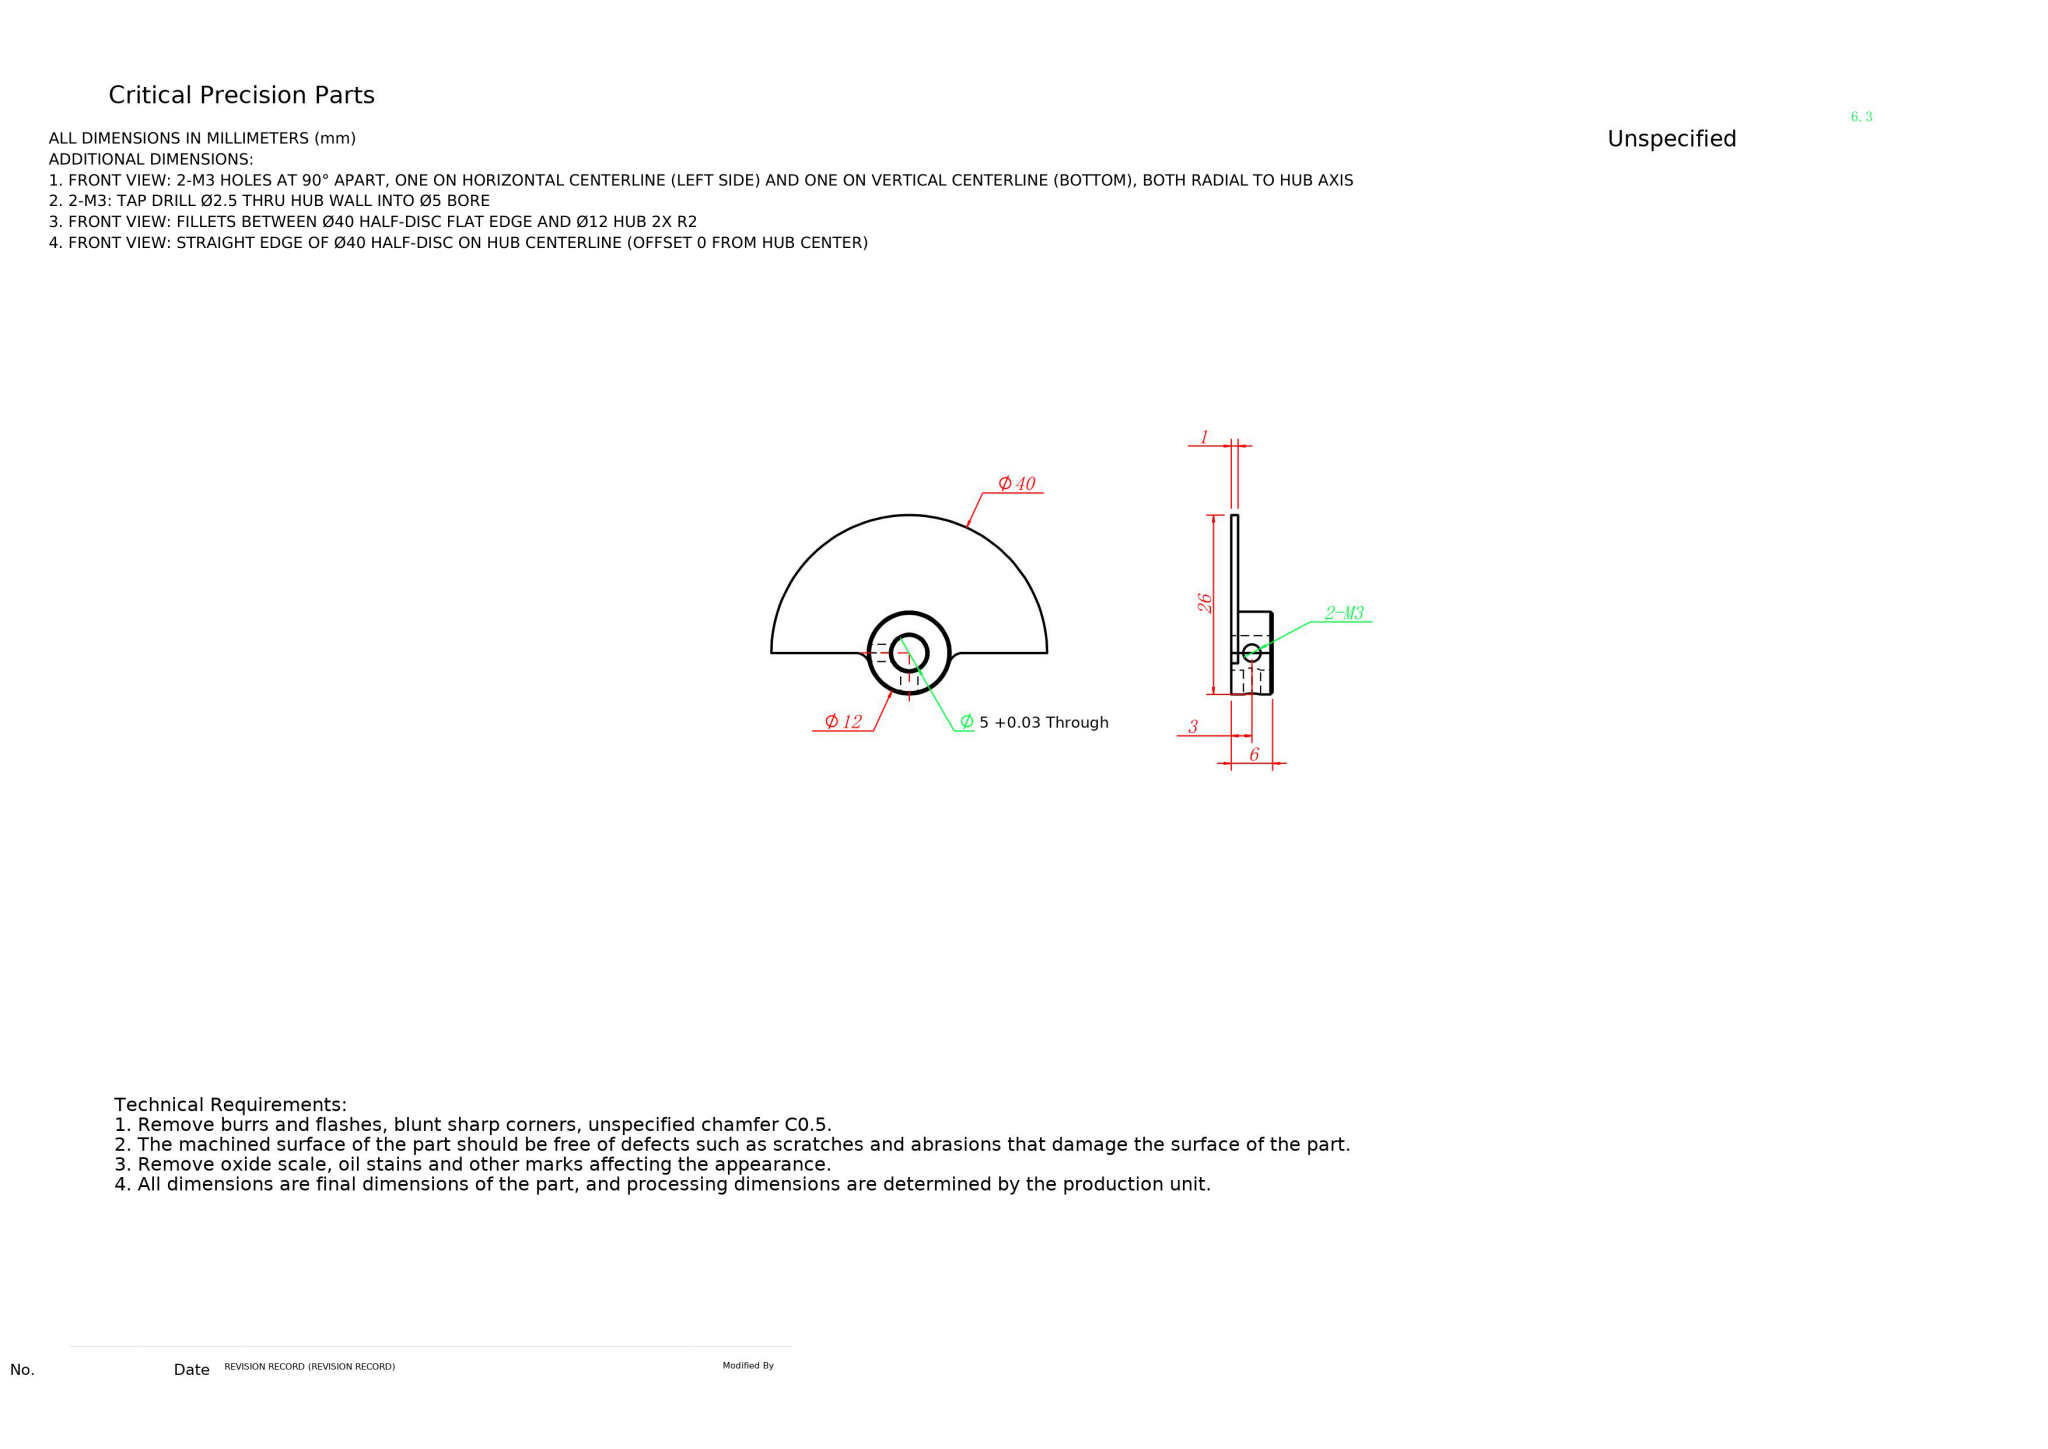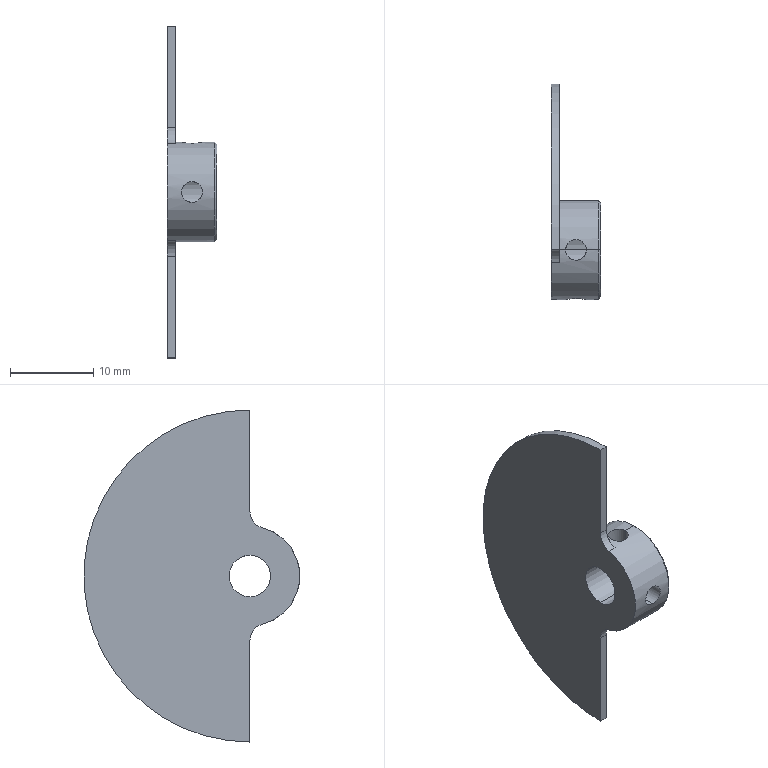Part | NX | mm | 1 solid | 22 faces | box 6 x 26 x 40 mm | volume 1096 mm3 | cylinder 13 | plane 5 | cone 4 | commonest cylinder face diameters 2.5 x4 1 x2 5 x2 12 x2 4 x2 40 x1
STEP:
#1=COLOUR_RGB('',0.7922,0.8196,0.9333);
#2=FILL_AREA_STYLE_COLOUR('',#1);
#3=FILL_AREA_STYLE('',(#2));
#4=SURFACE_STYLE_FILL_AREA(#3);
#5=SURFACE_SIDE_STYLE('',(#4));
#6=SURFACE_STYLE_USAGE(.BOTH.,#5);
#7=PRESENTATION_STYLE_ASSIGNMENT((#6));
#8=CARTESIAN_POINT('',(0.5,0.00003908,20.));
#9=VERTEX_POINT('',#8);
#10=CARTESIAN_POINT('',(0.5,-0.,19.994));
#11=VERTEX_POINT('',#10);
#12=CARTESIAN_POINT('',(0.5,0.5,19.994));
#13=DIRECTION('',(1.,0.,0.));
#14=DIRECTION('',(0.,0.,-1.));
#15=AXIS2_PLACEMENT_3D('',#12,#13,#14);
#16=CIRCLE('',#15,0.5);
#17=EDGE_CURVE('',#9,#11,#16,.T.);
#18=ORIENTED_EDGE('',*,*,#17,.F.);
#19=CARTESIAN_POINT('',(-0.5,0.00003908,20.));
#20=VERTEX_POINT('',#19);
#21=CARTESIAN_POINT('',(-0.0000125,0.00003908,20.));
#22=DIRECTION('',(-1.,0.,0.));
#23=VECTOR('',#22,1000.);
#24=LINE('',#21,#23);
#25=EDGE_CURVE('',#9,#20,#24,.T.);
#26=ORIENTED_EDGE('',*,*,#25,.T.);
#27=CARTESIAN_POINT('',(-0.5,-0.,19.994));
#28=VERTEX_POINT('',#27);
#29=CARTESIAN_POINT('',(-0.5,0.5,19.994));
#30=DIRECTION('',(-1.,0.,0.));
#31=DIRECTION('',(0.,0.,-1.));
#32=AXIS2_PLACEMENT_3D('',#29,#30,#31);
#33=CIRCLE('',#32,0.5);
#34=EDGE_CURVE('',#28,#20,#33,.T.);
#35=ORIENTED_EDGE('',*,*,#34,.F.);
#36=CARTESIAN_POINT('',(-0.5,-0.,19.994));
#37=DIRECTION('',(-1.,0.,0.));
#38=VECTOR('',#37,1000.);
#39=LINE('',#36,#38);
#40=EDGE_CURVE('',#11,#28,#39,.T.);
#41=ORIENTED_EDGE('',*,*,#40,.F.);
#42=EDGE_LOOP('',(#18,#26,#35,#41));
#43=FACE_OUTER_BOUND('',#42,.T.);
#44=CARTESIAN_POINT('',(0.5,0.5,19.994));
#45=DIRECTION('',(-1.,0.,0.));
#46=DIRECTION('',(0.,0.,1.));
#47=AXIS2_PLACEMENT_3D('',#44,#45,#46);
#48=CYLINDRICAL_SURFACE('',#47,0.5);
#49=ADVANCED_FACE('',(#43),#48,.T.);
#50=CARTESIAN_POINT('',(0.5,-0.,-19.994));
#51=VERTEX_POINT('',#50);
#52=CARTESIAN_POINT('',(0.5,0.00003908,-20.));
#53=VERTEX_POINT('',#52);
#54=CARTESIAN_POINT('',(0.5,0.5,-19.994));
#55=DIRECTION('',(1.,0.,0.));
#56=DIRECTION('',(0.,0.,-1.));
#57=AXIS2_PLACEMENT_3D('',#54,#55,#56);
#58=CIRCLE('',#57,0.5);
#59=EDGE_CURVE('',#51,#53,#58,.T.);
#60=ORIENTED_EDGE('',*,*,#59,.T.);
#61=CARTESIAN_POINT('',(0.5,0.,0.));
#62=DIRECTION('',(1.,0.,0.));
#63=DIRECTION('',(0.,0.,-1.));
#64=AXIS2_PLACEMENT_3D('',#61,#62,#63);
#65=CIRCLE('',#64,20.);
#66=EDGE_CURVE('',#53,#9,#65,.T.);
#67=ORIENTED_EDGE('',*,*,#66,.T.);
#68=ORIENTED_EDGE('',*,*,#17,.T.);
#69=CARTESIAN_POINT('',(0.5,-0.,7.746));
#70=VERTEX_POINT('',#69);
#71=CARTESIAN_POINT('',(0.5,0.,6.));
#72=DIRECTION('',(0.,-0.,1.));
#73=VECTOR('',#72,1000.);
#74=LINE('',#71,#73);
#75=EDGE_CURVE('',#70,#11,#74,.T.);
#76=ORIENTED_EDGE('',*,*,#75,.F.);
#77=CARTESIAN_POINT('',(0.5,-1.5,5.809));
#78=VERTEX_POINT('',#77);
#79=CARTESIAN_POINT('',(0.5,-2.,7.746));
#80=DIRECTION('',(-1.,0.,0.));
#81=DIRECTION('',(0.,0.,-1.));
#82=AXIS2_PLACEMENT_3D('',#79,#80,#81);
#83=CIRCLE('',#82,2.);
#84=EDGE_CURVE('',#70,#78,#83,.T.);
#85=ORIENTED_EDGE('',*,*,#84,.T.);
#86=CARTESIAN_POINT('',(0.5,0.,6.));
#87=VERTEX_POINT('',#86);
#88=CARTESIAN_POINT('',(0.5,0.,0.));
#89=DIRECTION('',(1.,0.,0.));
#90=DIRECTION('',(0.,0.,-1.));
#91=AXIS2_PLACEMENT_3D('',#88,#89,#90);
#92=CIRCLE('',#91,6.);
#93=EDGE_CURVE('',#87,#78,#92,.T.);
#94=ORIENTED_EDGE('',*,*,#93,.F.);
#95=CARTESIAN_POINT('',(0.5,0.,-6.));
#96=VERTEX_POINT('',#95);
#97=CARTESIAN_POINT('',(0.5,0.,0.));
#98=DIRECTION('',(1.,0.,0.));
#99=DIRECTION('',(0.,0.,-1.));
#100=AXIS2_PLACEMENT_3D('',#97,#98,#99);
#101=CIRCLE('',#100,6.);
#102=EDGE_CURVE('',#96,#87,#101,.T.);
#103=ORIENTED_EDGE('',*,*,#102,.F.);
#104=CARTESIAN_POINT('',(0.5,-1.5,-5.809));
#105=VERTEX_POINT('',#104);
#106=CARTESIAN_POINT('',(0.5,0.,0.));
#107=DIRECTION('',(1.,0.,0.));
#108=DIRECTION('',(0.,0.,-1.));
#109=AXIS2_PLACEMENT_3D('',#106,#107,#108);
#110=CIRCLE('',#109,6.);
#111=EDGE_CURVE('',#105,#96,#110,.T.);
#112=ORIENTED_EDGE('',*,*,#111,.F.);
#113=CARTESIAN_POINT('',(0.5,-0.,-7.746));
#114=VERTEX_POINT('',#113);
#115=CARTESIAN_POINT('',(0.5,-2.,-7.746));
#116=DIRECTION('',(-1.,0.,0.));
#117=DIRECTION('',(0.,0.,-1.));
#118=AXIS2_PLACEMENT_3D('',#115,#116,#117);
#119=CIRCLE('',#118,2.);
#120=EDGE_CURVE('',#105,#114,#119,.T.);
#121=ORIENTED_EDGE('',*,*,#120,.T.);
#122=CARTESIAN_POINT('',(0.5,-0.,-20.5));
#123=DIRECTION('',(0.,0.,1.));
#124=VECTOR('',#123,1000.);
#125=LINE('',#122,#124);
#126=EDGE_CURVE('',#51,#114,#125,.T.);
#127=ORIENTED_EDGE('',*,*,#126,.F.);
#128=EDGE_LOOP('',(#60,#67,#68,#76,#85,#94,#103,#112,#121,#127));
#129=FACE_OUTER_BOUND('',#128,.T.);
#130=CARTESIAN_POINT('',(0.5,0.,0.));
#131=DIRECTION('',(1.,0.,0.));
#132=DIRECTION('',(0.,1.,0.));
#133=AXIS2_PLACEMENT_3D('',#130,#131,#132);
#134=PLANE('',#133);
#135=ADVANCED_FACE('',(#129),#134,.T.);
#136=CARTESIAN_POINT('',(-0.5,0.,-2.5));
#137=VERTEX_POINT('',#136);
#138=CARTESIAN_POINT('',(-0.5,0.,2.5));
#139=VERTEX_POINT('',#138);
#140=CARTESIAN_POINT('',(-0.5,0.,0.));
#141=DIRECTION('',(1.,0.,0.));
#142=DIRECTION('',(0.,0.,-1.));
#143=AXIS2_PLACEMENT_3D('',#140,#141,#142);
#144=CIRCLE('',#143,2.5);
#145=EDGE_CURVE('',#137,#139,#144,.T.);
#146=ORIENTED_EDGE('',*,*,#145,.T.);
#147=CARTESIAN_POINT('',(-0.5,0.,0.));
#148=DIRECTION('',(1.,0.,0.));
#149=DIRECTION('',(0.,0.,-1.));
#150=AXIS2_PLACEMENT_3D('',#147,#148,#149);
#151=CIRCLE('',#150,2.5);
#152=EDGE_CURVE('',#139,#137,#151,.T.);
#153=ORIENTED_EDGE('',*,*,#152,.T.);
#154=EDGE_LOOP('',(#146,#153));
#155=FACE_BOUND('',#154,.T.);
#156=CARTESIAN_POINT('',(-0.5,0.00003908,-20.));
#157=VERTEX_POINT('',#156);
#158=CARTESIAN_POINT('',(-0.5,0.,0.));
#159=DIRECTION('',(1.,0.,0.));
#160=DIRECTION('',(0.,0.,-1.));
#161=AXIS2_PLACEMENT_3D('',#158,#159,#160);
#162=CIRCLE('',#161,20.);
#163=EDGE_CURVE('',#157,#20,#162,.T.);
#164=ORIENTED_EDGE('',*,*,#163,.F.);
#165=CARTESIAN_POINT('',(-0.5,-0.,-19.994));
#166=VERTEX_POINT('',#165);
#167=CARTESIAN_POINT('',(-0.5,0.5,-19.994));
#168=DIRECTION('',(-1.,0.,0.));
#169=DIRECTION('',(0.,0.,-1.));
#170=AXIS2_PLACEMENT_3D('',#167,#168,#169);
#171=CIRCLE('',#170,0.5);
#172=EDGE_CURVE('',#157,#166,#171,.T.);
#173=ORIENTED_EDGE('',*,*,#172,.T.);
#174=CARTESIAN_POINT('',(-0.5,-0.,-7.746));
#175=VERTEX_POINT('',#174);
#176=CARTESIAN_POINT('',(-0.5,-0.,-20.5));
#177=DIRECTION('',(0.,0.,1.));
#178=VECTOR('',#177,1000.);
#179=LINE('',#176,#178);
#180=EDGE_CURVE('',#166,#175,#179,.T.);
#181=ORIENTED_EDGE('',*,*,#180,.T.);
#182=CARTESIAN_POINT('',(-0.5,-1.5,-5.809));
#183=VERTEX_POINT('',#182);
#184=CARTESIAN_POINT('',(-0.5,-2.,-7.746));
#185=DIRECTION('',(1.,0.,0.));
#186=DIRECTION('',(0.,0.,-1.));
#187=AXIS2_PLACEMENT_3D('',#184,#185,#186);
#188=CIRCLE('',#187,2.);
#189=EDGE_CURVE('',#175,#183,#188,.T.);
#190=ORIENTED_EDGE('',*,*,#189,.T.);
#191=CARTESIAN_POINT('',(-0.5,-1.5,5.809));
#192=VERTEX_POINT('',#191);
#193=CARTESIAN_POINT('',(-0.5,0.,0.));
#194=DIRECTION('',(-1.,0.,0.));
#195=DIRECTION('',(0.,0.,1.));
#196=AXIS2_PLACEMENT_3D('',#193,#194,#195);
#197=CIRCLE('',#196,6.);
#198=EDGE_CURVE('',#183,#192,#197,.T.);
#199=ORIENTED_EDGE('',*,*,#198,.T.);
#200=CARTESIAN_POINT('',(-0.5,-0.,7.746));
#201=VERTEX_POINT('',#200);
#202=CARTESIAN_POINT('',(-0.5,-2.,7.746));
#203=DIRECTION('',(1.,0.,0.));
#204=DIRECTION('',(0.,0.,-1.));
#205=AXIS2_PLACEMENT_3D('',#202,#203,#204);
#206=CIRCLE('',#205,2.);
#207=EDGE_CURVE('',#192,#201,#206,.T.);
#208=ORIENTED_EDGE('',*,*,#207,.T.);
#209=CARTESIAN_POINT('',(-0.5,0.,6.));
#210=DIRECTION('',(0.,-0.,1.));
#211=VECTOR('',#210,1000.);
#212=LINE('',#209,#211);
#213=EDGE_CURVE('',#201,#28,#212,.T.);
#214=ORIENTED_EDGE('',*,*,#213,.T.);
#215=ORIENTED_EDGE('',*,*,#34,.T.);
#216=EDGE_LOOP('',(#164,#173,#181,#190,#199,#208,#214,#215));
#217=FACE_OUTER_BOUND('',#216,.T.);
#218=CARTESIAN_POINT('',(-0.5,0.,0.));
#219=DIRECTION('',(1.,0.,0.));
#220=DIRECTION('',(0.,1.,0.));
#221=AXIS2_PLACEMENT_3D('',#218,#219,#220);
#222=PLANE('',#221);
#223=ADVANCED_FACE('',(#155,#217),#222,.F.);
#224=ORIENTED_EDGE('',*,*,#172,.F.);
#225=CARTESIAN_POINT('',(-0.0000125,0.00003908,-20.));
#226=DIRECTION('',(1.,0.,0.));
#227=VECTOR('',#226,1000.);
#228=LINE('',#225,#227);
#229=EDGE_CURVE('',#157,#53,#228,.T.);
#230=ORIENTED_EDGE('',*,*,#229,.T.);
#231=ORIENTED_EDGE('',*,*,#59,.F.);
#232=CARTESIAN_POINT('',(-0.5,-0.,-19.994));
#233=DIRECTION('',(1.,0.,0.));
#234=VECTOR('',#233,1000.);
#235=LINE('',#232,#234);
#236=EDGE_CURVE('',#166,#51,#235,.T.);
#237=ORIENTED_EDGE('',*,*,#236,.F.);
#238=EDGE_LOOP('',(#224,#230,#231,#237));
#239=FACE_OUTER_BOUND('',#238,.T.);
#240=CARTESIAN_POINT('',(0.5,0.5,-19.994));
#241=DIRECTION('',(-1.,0.,0.));
#242=DIRECTION('',(0.,0.,1.));
#243=AXIS2_PLACEMENT_3D('',#240,#241,#242);
#244=CYLINDRICAL_SURFACE('',#243,0.5);
#245=ADVANCED_FACE('',(#239),#244,.T.);
#246=CARTESIAN_POINT('',(5.2,0.,2.5));
#247=VERTEX_POINT('',#246);
#248=CARTESIAN_POINT('',(5.2,0.,-2.5));
#249=VERTEX_POINT('',#248);
#250=CARTESIAN_POINT('',(5.2,0.,0.));
#251=DIRECTION('',(1.,0.,0.));
#252=DIRECTION('',(0.,0.,-1.));
#253=AXIS2_PLACEMENT_3D('',#250,#251,#252);
#254=CIRCLE('',#253,2.5);
#255=EDGE_CURVE('',#247,#249,#254,.T.);
#256=ORIENTED_EDGE('',*,*,#255,.F.);
#257=CARTESIAN_POINT('',(5.5,0.,2.8));
#258=VERTEX_POINT('',#257);
#259=CARTESIAN_POINT('',(5.2,0.,2.5));
#260=DIRECTION('',(0.7071,0.,0.7071));
#261=VECTOR('',#260,1000.);
#262=LINE('',#259,#261);
#263=EDGE_CURVE('',#247,#258,#262,.T.);
#264=ORIENTED_EDGE('',*,*,#263,.T.);
#265=CARTESIAN_POINT('',(5.5,0.,-2.8));
#266=VERTEX_POINT('',#265);
#267=CARTESIAN_POINT('',(5.5,0.,0.));
#268=DIRECTION('',(-1.,0.,0.));
#269=DIRECTION('',(0.,0.,-1.));
#270=AXIS2_PLACEMENT_3D('',#267,#268,#269);
#271=CIRCLE('',#270,2.8);
#272=EDGE_CURVE('',#266,#258,#271,.T.);
#273=ORIENTED_EDGE('',*,*,#272,.F.);
#274=CARTESIAN_POINT('',(5.2,0.,-2.5));
#275=DIRECTION('',(0.7071,0.,-0.7071));
#276=VECTOR('',#275,1000.);
#277=LINE('',#274,#276);
#278=EDGE_CURVE('',#249,#266,#277,.T.);
#279=ORIENTED_EDGE('',*,*,#278,.F.);
#280=EDGE_LOOP('',(#256,#264,#273,#279));
#281=FACE_OUTER_BOUND('',#280,.T.);
#282=CARTESIAN_POINT('',(5.2,0.,0.));
#283=DIRECTION('',(1.,0.,0.));
#284=DIRECTION('',(0.,0.,-1.));
#285=AXIS2_PLACEMENT_3D('',#282,#283,#284);
#286=CONICAL_SURFACE('',#285,2.5,0.7854);
#287=ADVANCED_FACE('',(#281),#286,.F.);
#288=CARTESIAN_POINT('',(5.5,0.,-5.7));
#289=VERTEX_POINT('',#288);
#290=CARTESIAN_POINT('',(5.5,0.,5.7));
#291=VERTEX_POINT('',#290);
#292=CARTESIAN_POINT('',(5.5,0.,0.));
#293=DIRECTION('',(1.,0.,0.));
#294=DIRECTION('',(0.,0.,-1.));
#295=AXIS2_PLACEMENT_3D('',#292,#293,#294);
#296=CIRCLE('',#295,5.7);
#297=EDGE_CURVE('',#289,#291,#296,.T.);
#298=ORIENTED_EDGE('',*,*,#297,.F.);
#299=CARTESIAN_POINT('',(5.2,0.,-6.));
#300=VERTEX_POINT('',#299);
#301=CARTESIAN_POINT('',(5.5,0.,-5.7));
#302=DIRECTION('',(-0.7071,0.,-0.7071));
#303=VECTOR('',#302,1000.);
#304=LINE('',#301,#303);
#305=EDGE_CURVE('',#289,#300,#304,.T.);
#306=ORIENTED_EDGE('',*,*,#305,.T.);
#307=CARTESIAN_POINT('',(5.2,0.,6.));
#308=VERTEX_POINT('',#307);
#309=CARTESIAN_POINT('',(5.2,0.,0.));
#310=DIRECTION('',(-1.,0.,0.));
#311=DIRECTION('',(0.,0.,-1.));
#312=AXIS2_PLACEMENT_3D('',#309,#310,#311);
#313=CIRCLE('',#312,6.);
#314=EDGE_CURVE('',#308,#300,#313,.T.);
#315=ORIENTED_EDGE('',*,*,#314,.F.);
#316=CARTESIAN_POINT('',(5.5,0.,5.7));
#317=DIRECTION('',(-0.7071,0.,0.7071));
#318=VECTOR('',#317,1000.);
#319=LINE('',#316,#318);
#320=EDGE_CURVE('',#291,#308,#319,.T.);
#321=ORIENTED_EDGE('',*,*,#320,.F.);
#322=EDGE_LOOP('',(#298,#306,#315,#321));
#323=FACE_OUTER_BOUND('',#322,.T.);
#324=CARTESIAN_POINT('',(5.5,0.,0.));
#325=DIRECTION('',(-1.,0.,0.));
#326=DIRECTION('',(0.,0.,1.));
#327=AXIS2_PLACEMENT_3D('',#324,#325,#326);
#328=CONICAL_SURFACE('',#327,5.7,0.7854);
#329=ADVANCED_FACE('',(#323),#328,.T.);
#330=CARTESIAN_POINT('',(2.5,-5.868,-1.25));
#331=VERTEX_POINT('',#330);
#332=CARTESIAN_POINT('',(2.5,-5.868,1.25));
#333=VERTEX_POINT('',#332);
#334=CARTESIAN_POINT('',(2.5,-5.868,-1.25));
#335=CARTESIAN_POINT('',(2.334,-5.868,-1.25));
#336=CARTESIAN_POINT('',(2.173,-5.875,-1.218));
#337=CARTESIAN_POINT('',(1.868,-5.9,-1.091));
#338=CARTESIAN_POINT('',(1.733,-5.917,-1.001));
#339=CARTESIAN_POINT('',(1.499,-5.952,-0.7671));
#340=CARTESIAN_POINT('',(1.41,-5.968,-0.6334));
#341=CARTESIAN_POINT('',(1.282,-5.993,-0.3259));
#342=CARTESIAN_POINT('',(1.25,-6.,-0.1652));
#343=CARTESIAN_POINT('',(1.25,-6.,0.1668));
#344=CARTESIAN_POINT('',(1.282,-5.993,0.3274));
#345=CARTESIAN_POINT('',(1.409,-5.968,0.6329));
#346=CARTESIAN_POINT('',(1.5,-5.952,0.7675));
#347=CARTESIAN_POINT('',(1.734,-5.917,1.002));
#348=CARTESIAN_POINT('',(1.868,-5.9,1.091));
#349=CARTESIAN_POINT('',(2.175,-5.875,1.218));
#350=CARTESIAN_POINT('',(2.334,-5.868,1.25));
#351=CARTESIAN_POINT('',(2.5,-5.868,1.25));
#352=B_SPLINE_CURVE_WITH_KNOTS('',3,(#334,#335,#336,#337,#338,#339,#340,#341,#342,#343,#344,#345,#346,#347,#348,#349,#350,#351),.UNSPECIFIED.,.F.,.F.,(4,2,2,2,2,2,2,2,4),(0.,0.125,0.25,0.375,0.5,0.625,0.75,0.875,1.),.UNSPECIFIED.);
#353=EDGE_CURVE('',#331,#333,#352,.T.);
#354=ORIENTED_EDGE('',*,*,#353,.F.);
#355=CARTESIAN_POINT('',(2.5,-2.165,-1.25));
#356=VERTEX_POINT('',#355);
#357=CARTESIAN_POINT('',(2.5,0.,-1.25));
#358=DIRECTION('',(0.,1.,0.));
#359=VECTOR('',#358,1000.);
#360=LINE('',#357,#359);
#361=EDGE_CURVE('',#331,#356,#360,.T.);
#362=ORIENTED_EDGE('',*,*,#361,.T.);
#363=CARTESIAN_POINT('',(2.5,-2.165,1.25));
#364=VERTEX_POINT('',#363);
#365=CARTESIAN_POINT('',(2.5,-2.165,1.25));
#366=CARTESIAN_POINT('',(2.417,-2.165,1.25));
#367=CARTESIAN_POINT('',(2.335,-2.17,1.242));
#368=CARTESIAN_POINT('',(2.214,-2.183,1.218));
#369=CARTESIAN_POINT('',(2.174,-2.189,1.208));
#370=CARTESIAN_POINT('',(2.095,-2.202,1.183));
#371=CARTESIAN_POINT('',(2.054,-2.21,1.168));
#372=CARTESIAN_POINT('',(1.942,-2.235,1.122));
#373=CARTESIAN_POINT('',(1.872,-2.253,1.084));
#374=CARTESIAN_POINT('',(1.738,-2.294,0.9946));
#375=CARTESIAN_POINT('',(1.674,-2.317,0.9421));
#376=CARTESIAN_POINT('',(1.559,-2.36,0.8264));
#377=CARTESIAN_POINT('',(1.507,-2.381,0.7641));
#378=CARTESIAN_POINT('',(1.417,-2.42,0.6307));
#379=CARTESIAN_POINT('',(1.38,-2.438,0.5611));
#380=CARTESIAN_POINT('',(1.283,-2.483,0.3294));
#381=CARTESIAN_POINT('',(1.25,-2.5,0.168));
#382=CARTESIAN_POINT('',(1.25,-2.5,-0.08278));
#383=CARTESIAN_POINT('',(1.258,-2.496,-0.1652));
#384=CARTESIAN_POINT('',(1.291,-2.48,-0.3271));
#385=CARTESIAN_POINT('',(1.316,-2.468,-0.4082));
#386=CARTESIAN_POINT('',(1.411,-2.423,-0.6357));
#387=CARTESIAN_POINT('',(1.5,-2.382,-0.768));
#388=CARTESIAN_POINT('',(1.676,-2.316,-0.944));
#389=CARTESIAN_POINT('',(1.739,-2.294,-0.9954));
#390=CARTESIAN_POINT('',(1.839,-2.263,-1.062));
#391=CARTESIAN_POINT('',(1.874,-2.253,-1.083));
#392=CARTESIAN_POINT('',(1.944,-2.235,-1.12));
#393=CARTESIAN_POINT('',(1.979,-2.227,-1.137));
#394=CARTESIAN_POINT('',(2.174,-2.184,-1.218));
#395=CARTESIAN_POINT('',(2.334,-2.165,-1.25));
#396=CARTESIAN_POINT('',(2.5,-2.165,-1.25));
#397=B_SPLINE_CURVE_WITH_KNOTS('',3,(#365,#366,#367,#368,#369,#370,#371,#372,#373,#374,#375,#376,#377,#378,#379,#380,#381,#382,#383,#384,#385,#386,#387,#388,#389,#390,#391,#392,#393,#394,#395,#396),.UNSPECIFIED.,.F.,.F.,(4,2,2,2,2,2,2,2,2,2,2,2,2,2,2,4),(0.,0.0625,0.09375,0.125,0.1875,0.25,0.3125,0.375,0.5,0.5625,0.625,0.75,0.8125,0.8438,0.875,1.),.UNSPECIFIED.);
#398=EDGE_CURVE('',#364,#356,#397,.T.);
#399=ORIENTED_EDGE('',*,*,#398,.F.);
#400=CARTESIAN_POINT('',(2.5,0.,1.25));
#401=DIRECTION('',(0.,1.,0.));
#402=VECTOR('',#401,1000.);
#403=LINE('',#400,#402);
#404=EDGE_CURVE('',#333,#364,#403,.T.);
#405=ORIENTED_EDGE('',*,*,#404,.F.);
#406=EDGE_LOOP('',(#354,#362,#399,#405));
#407=FACE_OUTER_BOUND('',#406,.T.);
#408=CARTESIAN_POINT('',(2.5,0.,0.));
#409=DIRECTION('',(0.,1.,0.));
#410=DIRECTION('',(0.,0.,1.));
#411=AXIS2_PLACEMENT_3D('',#408,#409,#410);
#412=CYLINDRICAL_SURFACE('',#411,1.25);
#413=ADVANCED_FACE('',(#407),#412,.F.);
#414=CARTESIAN_POINT('',(3.75,0.,6.));
#415=VERTEX_POINT('',#414);
#416=CARTESIAN_POINT('',(1.25,0.,6.));
#417=VERTEX_POINT('',#416);
#418=CARTESIAN_POINT('',(3.75,0.,6.));
#419=CARTESIAN_POINT('',(3.75,-0.166,6.));
#420=CARTESIAN_POINT('',(3.718,-0.3267,5.993));
#421=CARTESIAN_POINT('',(3.591,-0.6323,5.969));
#422=CARTESIAN_POINT('',(3.501,-0.767,5.952));
#423=CARTESIAN_POINT('',(3.266,-1.001,5.917));
#424=CARTESIAN_POINT('',(3.133,-1.091,5.9));
#425=CARTESIAN_POINT('',(2.826,-1.218,5.875));
#426=CARTESIAN_POINT('',(2.666,-1.25,5.868));
#427=CARTESIAN_POINT('',(2.335,-1.25,5.868));
#428=CARTESIAN_POINT('',(2.174,-1.218,5.875));
#429=CARTESIAN_POINT('',(1.869,-1.091,5.9));
#430=CARTESIAN_POINT('',(1.733,-1.001,5.917));
#431=CARTESIAN_POINT('',(1.499,-0.7668,5.952));
#432=CARTESIAN_POINT('',(1.409,-0.6322,5.969));
#433=CARTESIAN_POINT('',(1.282,-0.3256,5.993));
#434=CARTESIAN_POINT('',(1.25,-0.1658,6.));
#435=CARTESIAN_POINT('',(1.25,0.,6.));
#436=B_SPLINE_CURVE_WITH_KNOTS('',3,(#418,#419,#420,#421,#422,#423,#424,#425,#426,#427,#428,#429,#430,#431,#432,#433,#434,#435),.UNSPECIFIED.,.F.,.F.,(4,2,2,2,2,2,2,2,4),(0.,0.125,0.25,0.375,0.5,0.625,0.75,0.875,1.),.UNSPECIFIED.);
#437=EDGE_CURVE('',#415,#417,#436,.T.);
#438=ORIENTED_EDGE('',*,*,#437,.F.);
#439=CARTESIAN_POINT('',(3.75,0.,2.5));
#440=VERTEX_POINT('',#439);
#441=CARTESIAN_POINT('',(3.75,0.,0.));
#442=DIRECTION('',(0.,0.,-1.));
#443=VECTOR('',#442,1000.);
#444=LINE('',#441,#443);
#445=EDGE_CURVE('',#415,#440,#444,.T.);
#446=ORIENTED_EDGE('',*,*,#445,.T.);
#447=CARTESIAN_POINT('',(1.25,0.,2.5));
#448=VERTEX_POINT('',#447);
#449=CARTESIAN_POINT('',(1.25,0.,2.5));
#450=CARTESIAN_POINT('',(1.25,-0.08347,2.5));
#451=CARTESIAN_POINT('',(1.258,-0.1658,2.496));
#452=CARTESIAN_POINT('',(1.291,-0.3274,2.48));
#453=CARTESIAN_POINT('',(1.316,-0.4083,2.468));
#454=CARTESIAN_POINT('',(1.411,-0.6354,2.423));
#455=CARTESIAN_POINT('',(1.5,-0.7675,2.383));
#456=CARTESIAN_POINT('',(1.676,-0.9436,2.316));
#457=CARTESIAN_POINT('',(1.739,-0.9949,2.294));
#458=CARTESIAN_POINT('',(1.839,-1.062,2.263));
#459=CARTESIAN_POINT('',(1.873,-1.082,2.254));
#460=CARTESIAN_POINT('',(1.943,-1.12,2.235));
#461=CARTESIAN_POINT('',(1.978,-1.136,2.227));
#462=CARTESIAN_POINT('',(2.173,-1.218,2.184));
#463=CARTESIAN_POINT('',(2.333,-1.25,2.165));
#464=CARTESIAN_POINT('',(2.582,-1.25,2.165));
#465=CARTESIAN_POINT('',(2.664,-1.242,2.17));
#466=CARTESIAN_POINT('',(2.785,-1.218,2.183));
#467=CARTESIAN_POINT('',(2.825,-1.208,2.189));
#468=CARTESIAN_POINT('',(2.904,-1.184,2.202));
#469=CARTESIAN_POINT('',(2.946,-1.169,2.21));
#470=CARTESIAN_POINT('',(3.058,-1.122,2.235));
#471=CARTESIAN_POINT('',(3.128,-1.084,2.253));
#472=CARTESIAN_POINT('',(3.262,-0.9945,2.294));
#473=CARTESIAN_POINT('',(3.326,-0.9419,2.317));
#474=CARTESIAN_POINT('',(3.442,-0.826,2.36));
#475=CARTESIAN_POINT('',(3.493,-0.7637,2.382));
#476=CARTESIAN_POINT('',(3.583,-0.6301,2.42));
#477=CARTESIAN_POINT('',(3.62,-0.5604,2.438));
#478=CARTESIAN_POINT('',(3.718,-0.3286,2.483));
#479=CARTESIAN_POINT('',(3.75,-0.1667,2.5));
#480=CARTESIAN_POINT('',(3.75,0.,2.5));
#481=B_SPLINE_CURVE_WITH_KNOTS('',3,(#449,#450,#451,#452,#453,#454,#455,#456,#457,#458,#459,#460,#461,#462,#463,#464,#465,#466,#467,#468,#469,#470,#471,#472,#473,#474,#475,#476,#477,#478,#479,#480),.UNSPECIFIED.,.F.,.F.,(4,2,2,2,2,2,2,2,2,2,2,2,2,2,2,4),(0.,0.0625,0.125,0.25,0.3125,0.3438,0.375,0.5,0.5625,0.5938,0.625,0.6875,0.75,0.8125,0.875,1.),.UNSPECIFIED.);
#482=EDGE_CURVE('',#448,#440,#481,.T.);
#483=ORIENTED_EDGE('',*,*,#482,.F.);
#484=CARTESIAN_POINT('',(1.25,0.,0.));
#485=DIRECTION('',(0.,0.,-1.));
#486=VECTOR('',#485,1000.);
#487=LINE('',#484,#486);
#488=EDGE_CURVE('',#417,#448,#487,.T.);
#489=ORIENTED_EDGE('',*,*,#488,.F.);
#490=EDGE_LOOP('',(#438,#446,#483,#489));
#491=FACE_OUTER_BOUND('',#490,.T.);
#492=CARTESIAN_POINT('',(2.5,0.,0.));
#493=DIRECTION('',(0.,0.,-1.));
#494=DIRECTION('',(-1.,0.,0.));
#495=AXIS2_PLACEMENT_3D('',#492,#493,#494);
#496=CYLINDRICAL_SURFACE('',#495,1.25);
#497=ADVANCED_FACE('',(#491),#496,.F.);
#498=ORIENTED_EDGE('',*,*,#152,.F.);
#499=CARTESIAN_POINT('',(-0.5,0.,2.5));
#500=DIRECTION('',(1.,0.,0.));
#501=VECTOR('',#500,1000.);
#502=LINE('',#499,#501);
#503=EDGE_CURVE('',#139,#448,#502,.T.);
#504=ORIENTED_EDGE('',*,*,#503,.T.);
#505=ORIENTED_EDGE('',*,*,#482,.T.);
#506=CARTESIAN_POINT('',(-0.5,0.,2.5));
#507=DIRECTION('',(1.,0.,0.));
#508=VECTOR('',#507,1000.);
#509=LINE('',#506,#508);
#510=EDGE_CURVE('',#440,#247,#509,.T.);
#511=ORIENTED_EDGE('',*,*,#510,.T.);
#512=ORIENTED_EDGE('',*,*,#255,.T.);
#513=CARTESIAN_POINT('',(-0.5,0.,-2.5));
#514=DIRECTION('',(1.,0.,0.));
#515=VECTOR('',#514,1000.);
#516=LINE('',#513,#515);
#517=EDGE_CURVE('',#137,#249,#516,.T.);
#518=ORIENTED_EDGE('',*,*,#517,.F.);
#519=EDGE_LOOP('',(#498,#504,#505,#511,#512,#518));
#520=FACE_OUTER_BOUND('',#519,.T.);
#521=ORIENTED_EDGE('',*,*,#398,.T.);
#522=CARTESIAN_POINT('',(2.5,-2.165,-1.25));
#523=CARTESIAN_POINT('',(2.583,-2.165,-1.25));
#524=CARTESIAN_POINT('',(2.665,-2.17,-1.242));
#525=CARTESIAN_POINT('',(2.786,-2.183,-1.218));
#526=CARTESIAN_POINT('',(2.825,-2.189,-1.208));
#527=CARTESIAN_POINT('',(2.905,-2.202,-1.183));
#528=CARTESIAN_POINT('',(2.946,-2.21,-1.168));
#529=CARTESIAN_POINT('',(3.058,-2.235,-1.122));
#530=CARTESIAN_POINT('',(3.129,-2.253,-1.084));
#531=CARTESIAN_POINT('',(3.262,-2.294,-0.9945));
#532=CARTESIAN_POINT('',(3.326,-2.317,-0.9418));
#533=CARTESIAN_POINT('',(3.442,-2.36,-0.8261));
#534=CARTESIAN_POINT('',(3.493,-2.381,-0.7638));
#535=CARTESIAN_POINT('',(3.583,-2.42,-0.6303));
#536=CARTESIAN_POINT('',(3.62,-2.438,-0.5607));
#537=CARTESIAN_POINT('',(3.717,-2.483,-0.3292));
#538=CARTESIAN_POINT('',(3.75,-2.5,-0.1679));
#539=CARTESIAN_POINT('',(3.75,-2.5,0.08232));
#540=CARTESIAN_POINT('',(3.742,-2.496,0.1646));
#541=CARTESIAN_POINT('',(3.71,-2.48,0.3261));
#542=CARTESIAN_POINT('',(3.685,-2.468,0.4068));
#543=CARTESIAN_POINT('',(3.59,-2.423,0.6345));
#544=CARTESIAN_POINT('',(3.501,-2.383,0.767));
#545=CARTESIAN_POINT('',(3.324,-2.316,0.9433));
#546=CARTESIAN_POINT('',(3.262,-2.294,0.9948));
#547=CARTESIAN_POINT('',(3.162,-2.264,1.062));
#548=CARTESIAN_POINT('',(3.127,-2.254,1.082));
#549=CARTESIAN_POINT('',(3.057,-2.235,1.12));
#550=CARTESIAN_POINT('',(3.022,-2.227,1.136));
#551=CARTESIAN_POINT('',(2.827,-2.184,1.218));
#552=CARTESIAN_POINT('',(2.666,-2.165,1.25));
#553=CARTESIAN_POINT('',(2.5,-2.165,1.25));
#554=B_SPLINE_CURVE_WITH_KNOTS('',3,(#522,#523,#524,#525,#526,#527,#528,#529,#530,#531,#532,#533,#534,#535,#536,#537,#538,#539,#540,#541,#542,#543,#544,#545,#546,#547,#548,#549,#550,#551,#552,#553),.UNSPECIFIED.,.F.,.F.,(4,2,2,2,2,2,2,2,2,2,2,2,2,2,2,4),(0.,0.0625,0.09375,0.125,0.1875,0.25,0.3125,0.375,0.5,0.5625,0.625,0.75,0.8125,0.8437,0.875,1.),.UNSPECIFIED.);
#555=EDGE_CURVE('',#356,#364,#554,.T.);
#556=ORIENTED_EDGE('',*,*,#555,.T.);
#557=EDGE_LOOP('',(#521,#556));
#558=FACE_BOUND('',#557,.T.);
#559=CARTESIAN_POINT('',(-0.5,0.,0.));
#560=DIRECTION('',(1.,0.,0.));
#561=DIRECTION('',(0.,0.,-1.));
#562=AXIS2_PLACEMENT_3D('',#559,#560,#561);
#563=CYLINDRICAL_SURFACE('',#562,2.5);
#564=ADVANCED_FACE('',(#520,#558),#563,.F.);
#565=ORIENTED_EDGE('',*,*,#314,.T.);
#566=CARTESIAN_POINT('',(5.5,0.,-6.));
#567=DIRECTION('',(-1.,0.,0.));
#568=VECTOR('',#567,1000.);
#569=LINE('',#566,#568);
#570=EDGE_CURVE('',#300,#96,#569,.T.);
#571=ORIENTED_EDGE('',*,*,#570,.T.);
#572=ORIENTED_EDGE('',*,*,#102,.T.);
#573=CARTESIAN_POINT('',(5.5,0.,6.));
#574=DIRECTION('',(-1.,0.,0.));
#575=VECTOR('',#574,1000.);
#576=LINE('',#573,#575);
#577=EDGE_CURVE('',#417,#87,#576,.T.);
#578=ORIENTED_EDGE('',*,*,#577,.F.);
#579=CARTESIAN_POINT('',(1.25,0.,6.));
#580=CARTESIAN_POINT('',(1.25,0.1657,6.));
#581=CARTESIAN_POINT('',(1.282,0.326,5.993));
#582=CARTESIAN_POINT('',(1.409,0.6315,5.969));
#583=CARTESIAN_POINT('',(1.498,0.7661,5.952));
#584=CARTESIAN_POINT('',(1.733,1.001,5.917));
#585=CARTESIAN_POINT('',(1.867,1.09,5.9));
#586=CARTESIAN_POINT('',(2.174,1.218,5.875));
#587=CARTESIAN_POINT('',(2.334,1.25,5.868));
#588=CARTESIAN_POINT('',(2.665,1.25,5.868));
#589=CARTESIAN_POINT('',(2.826,1.218,5.875));
#590=CARTESIAN_POINT('',(3.131,1.092,5.9));
#591=CARTESIAN_POINT('',(3.266,1.001,5.917));
#592=CARTESIAN_POINT('',(3.5,0.7677,5.952));
#593=CARTESIAN_POINT('',(3.59,0.634,5.968));
#594=CARTESIAN_POINT('',(3.718,0.3266,5.993));
#595=CARTESIAN_POINT('',(3.75,0.1664,6.));
#596=CARTESIAN_POINT('',(3.75,0.,6.));
#597=B_SPLINE_CURVE_WITH_KNOTS('',3,(#579,#580,#581,#582,#583,#584,#585,#586,#587,#588,#589,#590,#591,#592,#593,#594,#595,#596),.UNSPECIFIED.,.F.,.F.,(4,2,2,2,2,2,2,2,4),(0.,0.125,0.25,0.375,0.5,0.625,0.75,0.875,1.),.UNSPECIFIED.);
#598=EDGE_CURVE('',#417,#415,#597,.T.);
#599=ORIENTED_EDGE('',*,*,#598,.T.);
#600=CARTESIAN_POINT('',(5.5,0.,6.));
#601=DIRECTION('',(-1.,0.,0.));
#602=VECTOR('',#601,1000.);
#603=LINE('',#600,#602);
#604=EDGE_CURVE('',#308,#415,#603,.T.);
#605=ORIENTED_EDGE('',*,*,#604,.F.);
#606=EDGE_LOOP('',(#565,#571,#572,#578,#599,#605));
#607=FACE_OUTER_BOUND('',#606,.T.);
#608=CARTESIAN_POINT('',(5.5,0.,0.));
#609=DIRECTION('',(-1.,0.,0.));
#610=DIRECTION('',(0.,0.,1.));
#611=AXIS2_PLACEMENT_3D('',#608,#609,#610);
#612=CYLINDRICAL_SURFACE('',#611,6.);
#613=ADVANCED_FACE('',(#607),#612,.T.);
#614=ORIENTED_EDGE('',*,*,#570,.F.);
#615=CARTESIAN_POINT('',(5.2,0.,0.));
#616=DIRECTION('',(-1.,0.,0.));
#617=DIRECTION('',(0.,0.,-1.));
#618=AXIS2_PLACEMENT_3D('',#615,#616,#617);
#619=CIRCLE('',#618,6.);
#620=EDGE_CURVE('',#300,#308,#619,.T.);
#621=ORIENTED_EDGE('',*,*,#620,.T.);
#622=ORIENTED_EDGE('',*,*,#604,.T.);
#623=ORIENTED_EDGE('',*,*,#437,.T.);
#624=ORIENTED_EDGE('',*,*,#577,.T.);
#625=ORIENTED_EDGE('',*,*,#93,.T.);
#626=CARTESIAN_POINT('',(5.5,-1.5,5.809));
#627=DIRECTION('',(-1.,0.,0.));
#628=VECTOR('',#627,1000.);
#629=LINE('',#626,#628);
#630=EDGE_CURVE('',#78,#192,#629,.T.);
#631=ORIENTED_EDGE('',*,*,#630,.T.);
#632=ORIENTED_EDGE('',*,*,#198,.F.);
#633=CARTESIAN_POINT('',(5.5,-1.5,-5.809));
#634=DIRECTION('',(1.,0.,0.));
#635=VECTOR('',#634,1000.);
#636=LINE('',#633,#635);
#637=EDGE_CURVE('',#183,#105,#636,.T.);
#638=ORIENTED_EDGE('',*,*,#637,.T.);
#639=ORIENTED_EDGE('',*,*,#111,.T.);
#640=EDGE_LOOP('',(#614,#621,#622,#623,#624,#625,#631,#632,#638,#639));
#641=FACE_OUTER_BOUND('',#640,.T.);
#642=CARTESIAN_POINT('',(2.5,-5.868,1.25));
#643=CARTESIAN_POINT('',(2.666,-5.868,1.25));
#644=CARTESIAN_POINT('',(2.826,-5.875,1.218));
#645=CARTESIAN_POINT('',(3.132,-5.9,1.091));
#646=CARTESIAN_POINT('',(3.267,-5.917,1.001));
#647=CARTESIAN_POINT('',(3.501,-5.952,0.7665));
#648=CARTESIAN_POINT('',(3.591,-5.969,0.6318));
#649=CARTESIAN_POINT('',(3.687,-5.987,0.4019));
#650=CARTESIAN_POINT('',(3.71,-5.992,0.3237));
#651=CARTESIAN_POINT('',(3.742,-5.998,0.164));
#652=CARTESIAN_POINT('',(3.75,-6.,0.0813));
#653=CARTESIAN_POINT('',(3.75,-6.,-0.08187));
#654=CARTESIAN_POINT('',(3.742,-5.998,-0.1635));
#655=CARTESIAN_POINT('',(3.71,-5.992,-0.3255));
#656=CARTESIAN_POINT('',(3.686,-5.987,-0.4027));
#657=CARTESIAN_POINT('',(3.591,-5.969,-0.6319));
#658=CARTESIAN_POINT('',(3.501,-5.952,-0.7664));
#659=CARTESIAN_POINT('',(3.267,-5.917,-1.001));
#660=CARTESIAN_POINT('',(3.133,-5.9,-1.091));
#661=CARTESIAN_POINT('',(2.826,-5.875,-1.218));
#662=CARTESIAN_POINT('',(2.666,-5.868,-1.25));
#663=CARTESIAN_POINT('',(2.5,-5.868,-1.25));
#664=B_SPLINE_CURVE_WITH_KNOTS('',3,(#642,#643,#644,#645,#646,#647,#648,#649,#650,#651,#652,#653,#654,#655,#656,#657,#658,#659,#660,#661,#662,#663),.UNSPECIFIED.,.F.,.F.,(4,2,2,2,2,2,2,2,2,2,4),(0.,0.125,0.25,0.375,0.4375,0.5,0.5625,0.625,0.75,0.875,1.),.UNSPECIFIED.);
#665=EDGE_CURVE('',#333,#331,#664,.T.);
#666=ORIENTED_EDGE('',*,*,#665,.T.);
#667=ORIENTED_EDGE('',*,*,#353,.T.);
#668=EDGE_LOOP('',(#666,#667));
#669=FACE_BOUND('',#668,.T.);
#670=CARTESIAN_POINT('',(5.5,0.,0.));
#671=DIRECTION('',(-1.,0.,0.));
#672=DIRECTION('',(0.,0.,1.));
#673=AXIS2_PLACEMENT_3D('',#670,#671,#672);
#674=CYLINDRICAL_SURFACE('',#673,6.);
#675=ADVANCED_FACE('',(#641,#669),#674,.T.);
#676=CARTESIAN_POINT('',(5.5,0.,0.));
#677=DIRECTION('',(1.,0.,0.));
#678=DIRECTION('',(0.,0.,-1.));
#679=AXIS2_PLACEMENT_3D('',#676,#677,#678);
#680=CIRCLE('',#679,5.7);
#681=EDGE_CURVE('',#291,#289,#680,.T.);
#682=ORIENTED_EDGE('',*,*,#681,.T.);
#683=ORIENTED_EDGE('',*,*,#297,.T.);
#684=EDGE_LOOP('',(#682,#683));
#685=FACE_OUTER_BOUND('',#684,.T.);
#686=ORIENTED_EDGE('',*,*,#272,.T.);
#687=CARTESIAN_POINT('',(5.5,0.,0.));
#688=DIRECTION('',(-1.,0.,0.));
#689=DIRECTION('',(0.,0.,-1.));
#690=AXIS2_PLACEMENT_3D('',#687,#688,#689);
#691=CIRCLE('',#690,2.8);
#692=EDGE_CURVE('',#258,#266,#691,.T.);
#693=ORIENTED_EDGE('',*,*,#692,.T.);
#694=EDGE_LOOP('',(#686,#693));
#695=FACE_BOUND('',#694,.T.);
#696=CARTESIAN_POINT('',(5.5,0.,0.));
#697=DIRECTION('',(1.,0.,0.));
#698=DIRECTION('',(0.,1.,0.));
#699=AXIS2_PLACEMENT_3D('',#696,#697,#698);
#700=PLANE('',#699);
#701=ADVANCED_FACE('',(#685,#695),#700,.T.);
#702=ORIENTED_EDGE('',*,*,#503,.F.);
#703=ORIENTED_EDGE('',*,*,#145,.F.);
#704=ORIENTED_EDGE('',*,*,#517,.T.);
#705=CARTESIAN_POINT('',(5.2,0.,0.));
#706=DIRECTION('',(1.,0.,0.));
#707=DIRECTION('',(0.,0.,-1.));
#708=AXIS2_PLACEMENT_3D('',#705,#706,#707);
#709=CIRCLE('',#708,2.5);
#710=EDGE_CURVE('',#249,#247,#709,.T.);
#711=ORIENTED_EDGE('',*,*,#710,.T.);
#712=ORIENTED_EDGE('',*,*,#510,.F.);
#713=CARTESIAN_POINT('',(3.75,0.,2.5));
#714=CARTESIAN_POINT('',(3.75,0.08344,2.5));
#715=CARTESIAN_POINT('',(3.742,0.1657,2.496));
#716=CARTESIAN_POINT('',(3.709,0.3272,2.48));
#717=CARTESIAN_POINT('',(3.684,0.408,2.468));
#718=CARTESIAN_POINT('',(3.589,0.6354,2.423));
#719=CARTESIAN_POINT('',(3.5,0.7678,2.382));
#720=CARTESIAN_POINT('',(3.324,0.9438,2.316));
#721=CARTESIAN_POINT('',(3.261,0.9951,2.294));
#722=CARTESIAN_POINT('',(3.161,1.062,2.263));
#723=CARTESIAN_POINT('',(3.127,1.082,2.254));
#724=CARTESIAN_POINT('',(3.056,1.12,2.235));
#725=CARTESIAN_POINT('',(3.022,1.137,2.227));
#726=CARTESIAN_POINT('',(2.827,1.218,2.184));
#727=CARTESIAN_POINT('',(2.667,1.25,2.165));
#728=CARTESIAN_POINT('',(2.419,1.25,2.165));
#729=CARTESIAN_POINT('',(2.337,1.242,2.17));
#730=CARTESIAN_POINT('',(2.216,1.218,2.183));
#731=CARTESIAN_POINT('',(2.176,1.208,2.189));
#732=CARTESIAN_POINT('',(2.097,1.184,2.202));
#733=CARTESIAN_POINT('',(2.056,1.169,2.21));
#734=CARTESIAN_POINT('',(1.943,1.122,2.234));
#735=CARTESIAN_POINT('',(1.873,1.084,2.253));
#736=CARTESIAN_POINT('',(1.739,0.9952,2.294));
#737=CARTESIAN_POINT('',(1.675,0.9426,2.316));
#738=CARTESIAN_POINT('',(1.559,0.8268,2.36));
#739=CARTESIAN_POINT('',(1.507,0.7645,2.381));
#740=CARTESIAN_POINT('',(1.418,0.631,2.42));
#741=CARTESIAN_POINT('',(1.38,0.5614,2.437));
#742=CARTESIAN_POINT('',(1.283,0.3293,2.483));
#743=CARTESIAN_POINT('',(1.25,0.167,2.5));
#744=CARTESIAN_POINT('',(1.25,0.,2.5));
#745=B_SPLINE_CURVE_WITH_KNOTS('',3,(#713,#714,#715,#716,#717,#718,#719,#720,#721,#722,#723,#724,#725,#726,#727,#728,#729,#730,#731,#732,#733,#734,#735,#736,#737,#738,#739,#740,#741,#742,#743,#744),.UNSPECIFIED.,.F.,.F.,(4,2,2,2,2,2,2,2,2,2,2,2,2,2,2,4),(0.,0.0625,0.125,0.25,0.3125,0.3437,0.375,0.5,0.5625,0.5937,0.625,0.6875,0.75,0.8125,0.875,1.),.UNSPECIFIED.);
#746=EDGE_CURVE('',#440,#448,#745,.T.);
#747=ORIENTED_EDGE('',*,*,#746,.T.);
#748=EDGE_LOOP('',(#702,#703,#704,#711,#712,#747));
#749=FACE_OUTER_BOUND('',#748,.T.);
#750=CARTESIAN_POINT('',(-0.5,0.,0.));
#751=DIRECTION('',(1.,0.,0.));
#752=DIRECTION('',(0.,0.,-1.));
#753=AXIS2_PLACEMENT_3D('',#750,#751,#752);
#754=CYLINDRICAL_SURFACE('',#753,2.5);
#755=ADVANCED_FACE('',(#749),#754,.F.);
#756=ORIENTED_EDGE('',*,*,#180,.F.);
#757=ORIENTED_EDGE('',*,*,#236,.T.);
#758=ORIENTED_EDGE('',*,*,#126,.T.);
#759=CARTESIAN_POINT('',(-0.5,-0.,-7.746));
#760=DIRECTION('',(-1.,0.,0.));
#761=VECTOR('',#760,1000.);
#762=LINE('',#759,#761);
#763=EDGE_CURVE('',#114,#175,#762,.T.);
#764=ORIENTED_EDGE('',*,*,#763,.T.);
#765=EDGE_LOOP('',(#756,#757,#758,#764));
#766=FACE_OUTER_BOUND('',#765,.T.);
#767=CARTESIAN_POINT('',(-0.5,-0.,-20.5));
#768=DIRECTION('',(0.,1.,-0.));
#769=DIRECTION('',(1.,0.,0.));
#770=AXIS2_PLACEMENT_3D('',#767,#768,#769);
#771=PLANE('',#770);
#772=ADVANCED_FACE('',(#766),#771,.F.);
#773=ORIENTED_EDGE('',*,*,#75,.T.);
#774=ORIENTED_EDGE('',*,*,#40,.T.);
#775=ORIENTED_EDGE('',*,*,#213,.F.);
#776=CARTESIAN_POINT('',(0.5,-0.,7.746));
#777=DIRECTION('',(1.,0.,0.));
#778=VECTOR('',#777,1000.);
#779=LINE('',#776,#778);
#780=EDGE_CURVE('',#201,#70,#779,.T.);
#781=ORIENTED_EDGE('',*,*,#780,.T.);
#782=EDGE_LOOP('',(#773,#774,#775,#781));
#783=FACE_OUTER_BOUND('',#782,.T.);
#784=CARTESIAN_POINT('',(-0.5,0.,6.));
#785=DIRECTION('',(0.,1.,0.));
#786=DIRECTION('',(1.,0.,0.));
#787=AXIS2_PLACEMENT_3D('',#784,#785,#786);
#788=PLANE('',#787);
#789=ADVANCED_FACE('',(#783),#788,.F.);
#790=ORIENTED_EDGE('',*,*,#445,.F.);
#791=ORIENTED_EDGE('',*,*,#598,.F.);
#792=ORIENTED_EDGE('',*,*,#488,.T.);
#793=ORIENTED_EDGE('',*,*,#746,.F.);
#794=EDGE_LOOP('',(#790,#791,#792,#793));
#795=FACE_OUTER_BOUND('',#794,.T.);
#796=CARTESIAN_POINT('',(2.5,0.,0.));
#797=DIRECTION('',(0.,0.,-1.));
#798=DIRECTION('',(-1.,0.,0.));
#799=AXIS2_PLACEMENT_3D('',#796,#797,#798);
#800=CYLINDRICAL_SURFACE('',#799,1.25);
#801=ADVANCED_FACE('',(#795),#800,.F.);
#802=ORIENTED_EDGE('',*,*,#361,.F.);
#803=ORIENTED_EDGE('',*,*,#665,.F.);
#804=ORIENTED_EDGE('',*,*,#404,.T.);
#805=ORIENTED_EDGE('',*,*,#555,.F.);
#806=EDGE_LOOP('',(#802,#803,#804,#805));
#807=FACE_OUTER_BOUND('',#806,.T.);
#808=CARTESIAN_POINT('',(2.5,0.,0.));
#809=DIRECTION('',(0.,1.,0.));
#810=DIRECTION('',(0.,0.,1.));
#811=AXIS2_PLACEMENT_3D('',#808,#809,#810);
#812=CYLINDRICAL_SURFACE('',#811,1.25);
#813=ADVANCED_FACE('',(#807),#812,.F.);
#814=ORIENTED_EDGE('',*,*,#207,.F.);
#815=ORIENTED_EDGE('',*,*,#630,.F.);
#816=ORIENTED_EDGE('',*,*,#84,.F.);
#817=ORIENTED_EDGE('',*,*,#780,.F.);
#818=EDGE_LOOP('',(#814,#815,#816,#817));
#819=FACE_OUTER_BOUND('',#818,.T.);
#820=CARTESIAN_POINT('',(5.5,-2.,7.746));
#821=DIRECTION('',(-1.,0.,0.));
#822=DIRECTION('',(0.,0.,1.));
#823=AXIS2_PLACEMENT_3D('',#820,#821,#822);
#824=CYLINDRICAL_SURFACE('',#823,2.);
#825=ADVANCED_FACE('',(#819),#824,.F.);
#826=ORIENTED_EDGE('',*,*,#189,.F.);
#827=ORIENTED_EDGE('',*,*,#763,.F.);
#828=ORIENTED_EDGE('',*,*,#120,.F.);
#829=ORIENTED_EDGE('',*,*,#637,.F.);
#830=EDGE_LOOP('',(#826,#827,#828,#829));
#831=FACE_OUTER_BOUND('',#830,.T.);
#832=CARTESIAN_POINT('',(5.5,-2.,-7.746));
#833=DIRECTION('',(-1.,0.,0.));
#834=DIRECTION('',(0.,0.,1.));
#835=AXIS2_PLACEMENT_3D('',#832,#833,#834);
#836=CYLINDRICAL_SURFACE('',#835,2.);
#837=ADVANCED_FACE('',(#831),#836,.F.);
#838=ORIENTED_EDGE('',*,*,#305,.F.);
#839=ORIENTED_EDGE('',*,*,#681,.F.);
#840=ORIENTED_EDGE('',*,*,#320,.T.);
#841=ORIENTED_EDGE('',*,*,#620,.F.);
#842=EDGE_LOOP('',(#838,#839,#840,#841));
#843=FACE_OUTER_BOUND('',#842,.T.);
#844=CARTESIAN_POINT('',(5.5,0.,0.));
#845=DIRECTION('',(-1.,0.,0.));
#846=DIRECTION('',(0.,0.,1.));
#847=AXIS2_PLACEMENT_3D('',#844,#845,#846);
#848=CONICAL_SURFACE('',#847,5.7,0.7854);
#849=ADVANCED_FACE('',(#843),#848,.T.);
#850=ORIENTED_EDGE('',*,*,#263,.F.);
#851=ORIENTED_EDGE('',*,*,#710,.F.);
#852=ORIENTED_EDGE('',*,*,#278,.T.);
#853=ORIENTED_EDGE('',*,*,#692,.F.);
#854=EDGE_LOOP('',(#850,#851,#852,#853));
#855=FACE_OUTER_BOUND('',#854,.T.);
#856=CARTESIAN_POINT('',(5.2,0.,0.));
#857=DIRECTION('',(1.,0.,0.));
#858=DIRECTION('',(0.,0.,-1.));
#859=AXIS2_PLACEMENT_3D('',#856,#857,#858);
#860=CONICAL_SURFACE('',#859,2.5,0.7854);
#861=ADVANCED_FACE('',(#855),#860,.F.);
#862=ORIENTED_EDGE('',*,*,#66,.F.);
#863=ORIENTED_EDGE('',*,*,#229,.F.);
#864=ORIENTED_EDGE('',*,*,#163,.T.);
#865=ORIENTED_EDGE('',*,*,#25,.F.);
#866=EDGE_LOOP('',(#862,#863,#864,#865));
#867=FACE_OUTER_BOUND('',#866,.T.);
#868=CARTESIAN_POINT('',(-0.5,0.,0.));
#869=DIRECTION('',(1.,0.,0.));
#870=DIRECTION('',(0.,0.,-1.));
#871=AXIS2_PLACEMENT_3D('',#868,#869,#870);
#872=CYLINDRICAL_SURFACE('',#871,20.);
#873=ADVANCED_FACE('',(#867),#872,.T.);
#874=CLOSED_SHELL('',(#49,#135,#223,#245,#287,#329,#413,#497,#564,#613,#675,#701,#755,#772,#789,#801,#813,#825,#837,#849,#861,#873));
#875=MANIFOLD_SOLID_BREP('',#874);
#876=STYLED_ITEM('',(#7),#875);
#877=PRESENTATION_LAYER_ASSIGNMENT('','',(#876));
#878=CARTESIAN_POINT('',(0.,0.,0.));
#879=DIRECTION('',(0.,0.,1.));
#880=DIRECTION('',(1.,0.,0.));
#881=AXIS2_PLACEMENT_3D('',#878,#879,#880);
#882=(LENGTH_UNIT()NAMED_UNIT(*)SI_UNIT(.MILLI.,.METRE.));
#883=UNCERTAINTY_MEASURE_WITH_UNIT(LENGTH_MEASURE(0.00001),#882,'','');
#884=(NAMED_UNIT(*)PLANE_ANGLE_UNIT()SI_UNIT($,.RADIAN.));
#885=(NAMED_UNIT(*)SI_UNIT($,.STERADIAN.)SOLID_ANGLE_UNIT());
#886=(GEOMETRIC_REPRESENTATION_CONTEXT(3)GLOBAL_UNCERTAINTY_ASSIGNED_CONTEXT((#883))GLOBAL_UNIT_ASSIGNED_CONTEXT((#882,#884,#885))REPRESENTATION_CONTEXT('',''));
#887=ADVANCED_BREP_SHAPE_REPRESENTATION('',(#875,#881),#886);
#888=(LENGTH_UNIT()NAMED_UNIT(*)SI_UNIT(.MILLI.,.METRE.));
#889=UNCERTAINTY_MEASURE_WITH_UNIT(LENGTH_MEASURE(0.00001),#888,'','');
#890=(NAMED_UNIT(*)PLANE_ANGLE_UNIT()SI_UNIT($,.RADIAN.));
#891=(NAMED_UNIT(*)SI_UNIT($,.STERADIAN.)SOLID_ANGLE_UNIT());
#892=(GEOMETRIC_REPRESENTATION_CONTEXT(3)GLOBAL_UNCERTAINTY_ASSIGNED_CONTEXT((#889))GLOBAL_UNIT_ASSIGNED_CONTEXT((#888,#890,#891))REPRESENTATION_CONTEXT('',''));
#893=MECHANICAL_DESIGN_GEOMETRIC_PRESENTATION_REPRESENTATION('',(#876),#892);